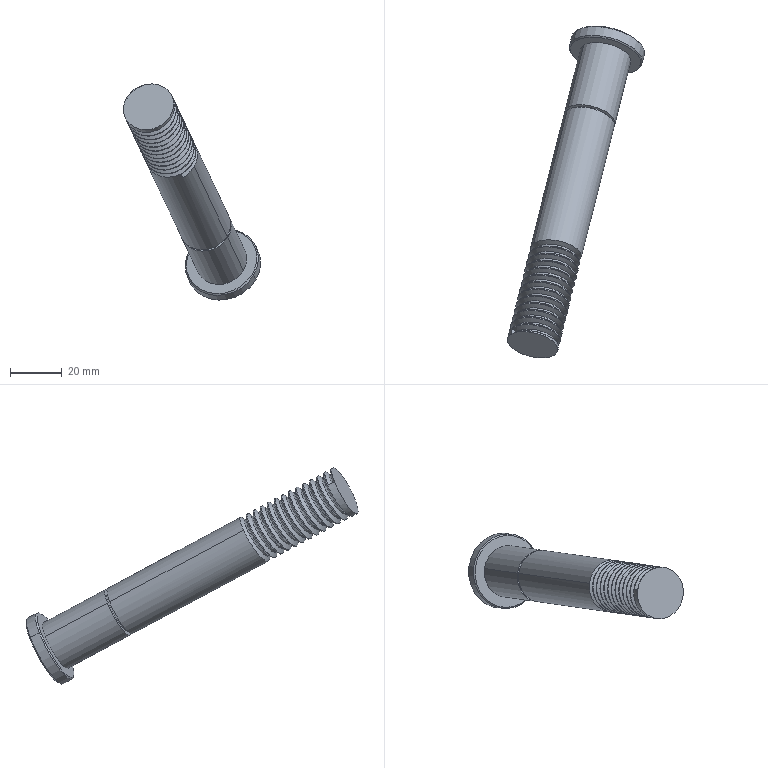Component | SolidWorks | ScribingMechanismAssembly-1_AttachedSoilDiskAssembly-1_AttachedSoilDiskAxis-1 | 1 solid | 47 faces | volume 41765 mm3 | cylinder 33 | plane 7 | cone 4 | spline 3 | commonest cylinder face diameters 20 x29 17 x2 29 x2